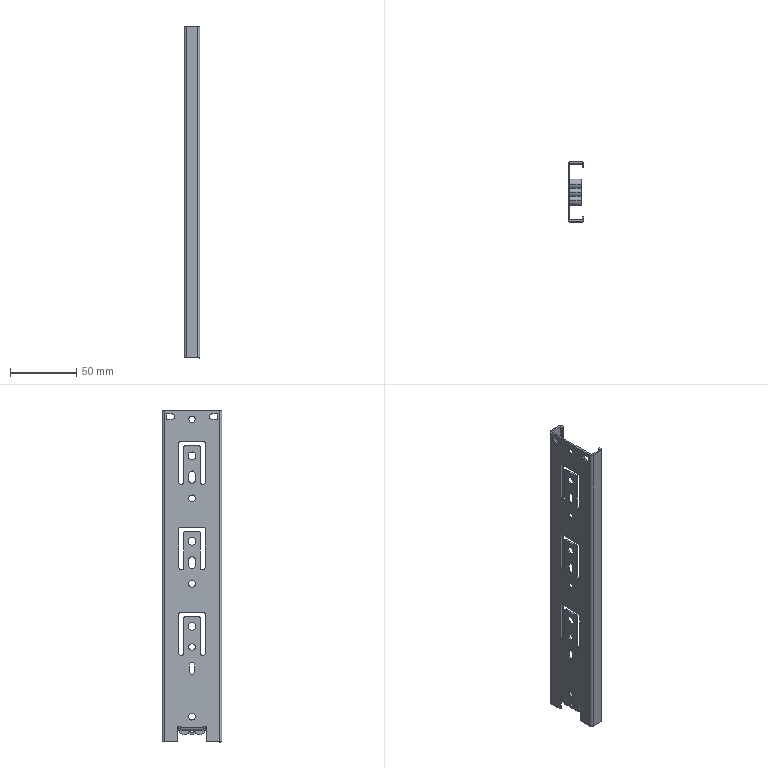Component | SolidWorks | PC-CAJ-P09-1_Corredera A 250-3 | 1 solid | 150 faces | volume 20190 mm3 | plane 83 | cylinder 67 | commonest cylinder face diameters 2 x12 8 x9 5 x8 4.7 x6 6 x6 3.8 x6 4 x5 1 x5 | material Plain Carbon Steel